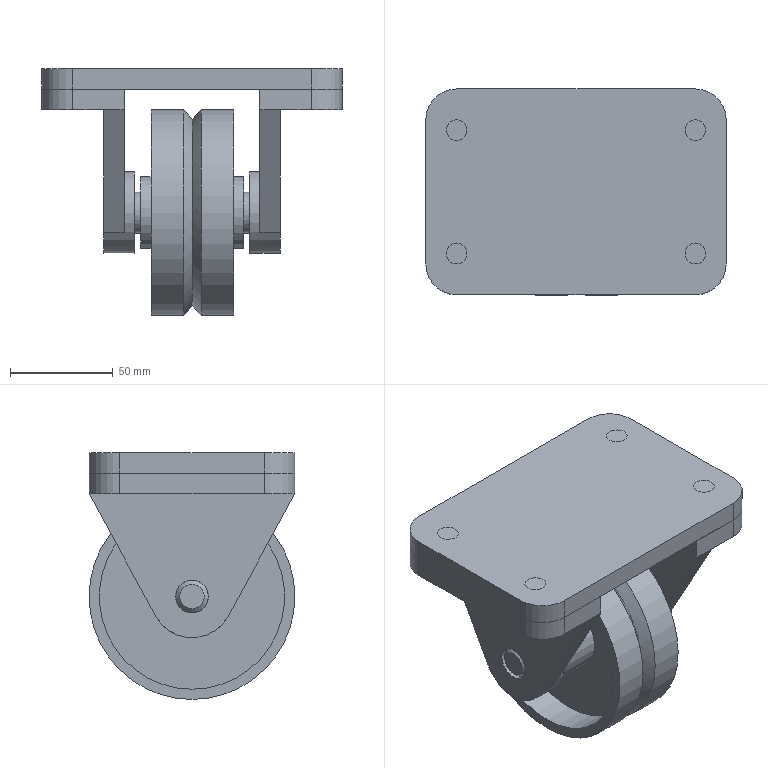Assembly | NX | mm | 9 component files | 9 solids | 82 faces | box 146 x 100 x 120 mm | volume 477283 mm3 | plane 44 | cylinder 34 | cone 4 | commonest cylinder face diameters 10 x12 30 x8 40 x2 16 x2 100 x2 90 x2 35 x2 15.9 x2
Bill of materials:
unnamed part 1 | 1 |  | Thin flat rectangular plate with rounded corners and four through-holes, one near each corner.
unnamed part 2 | 4 |  | Plain solid right circular cylinder, about twice as long as its diameter.
unnamed part 3 | 2 |  | L-shaped bracket: a flat top flange with two through-holes, and a tapered web below it that ends in a rounded lug with one larger through-hole and a raised boss on one side.
unnamed part 4 | 1 |  | Wheel with a V-shaped groove around its outer edge, recessed side faces, and a central hub with a through-bore that sticks out past both side faces.
unnamed part 5 | 1 |  | Solid stepped round pin: a larger-diameter middle section with a shorter, smaller-diameter journal at each end, and chamfered end faces.
Mates:
1. fix | base_100 1 component
2. fix | base_100 1 component
3. touch align | suporte_roda 2 face | base_100 1 face
4. touch align | suporte_roda 2 face | base_100 1 face
5. touch align | suporte_roda 2 face | base_100 1 face
6. touch align | suporte_roda 1 face | suporte_roda 2 face
7. touch align | suporte_roda 1 face | base_100 1 face
8. touch align | suporte_roda 1 face | base_100 1 face
9. touch align | roda_100 1 | suporte_roda 2 face
10. touch align | eixo_roda 1 face | suporte_roda 1 face
11. touch align | eixo_roda 1 face | suporte_roda 1 face
12. touch align | pino_base4furo 4 face | base_100 1 face
13. touch align | pino_base4furo 3 face | base_100 1 face
14. touch align | pino_base4furo 2 face | base_100 1 face
15. touch align | pino_base4furo 1 face | base_100 1 face